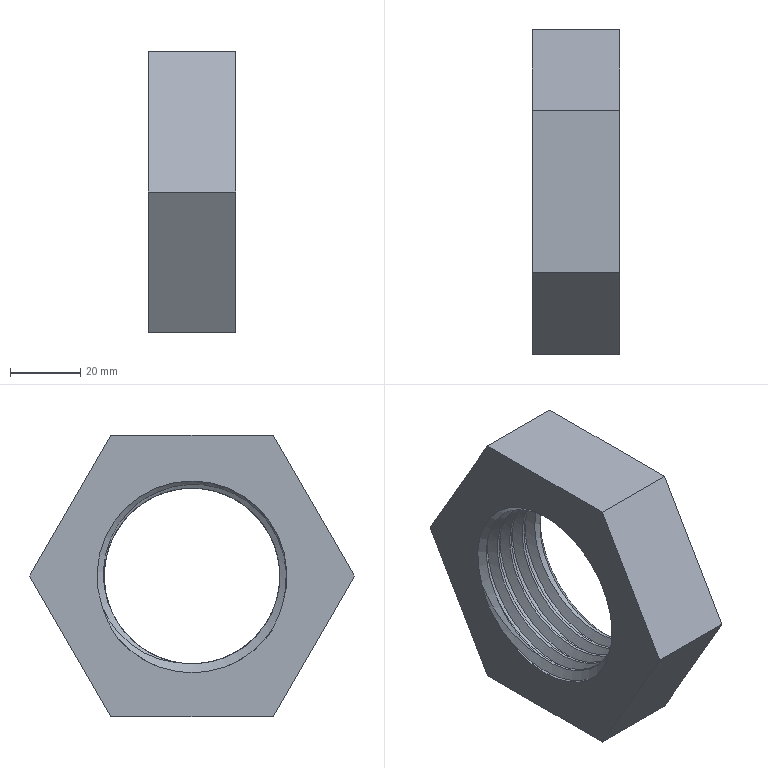Component | NX | PIN_NUT | 1 solid | 15 faces | volume 84150 mm3 | plane 9 | cylinder 2 | cone 2 | spline 2 | commonest cylinder face diameters 50 x1 55 x1